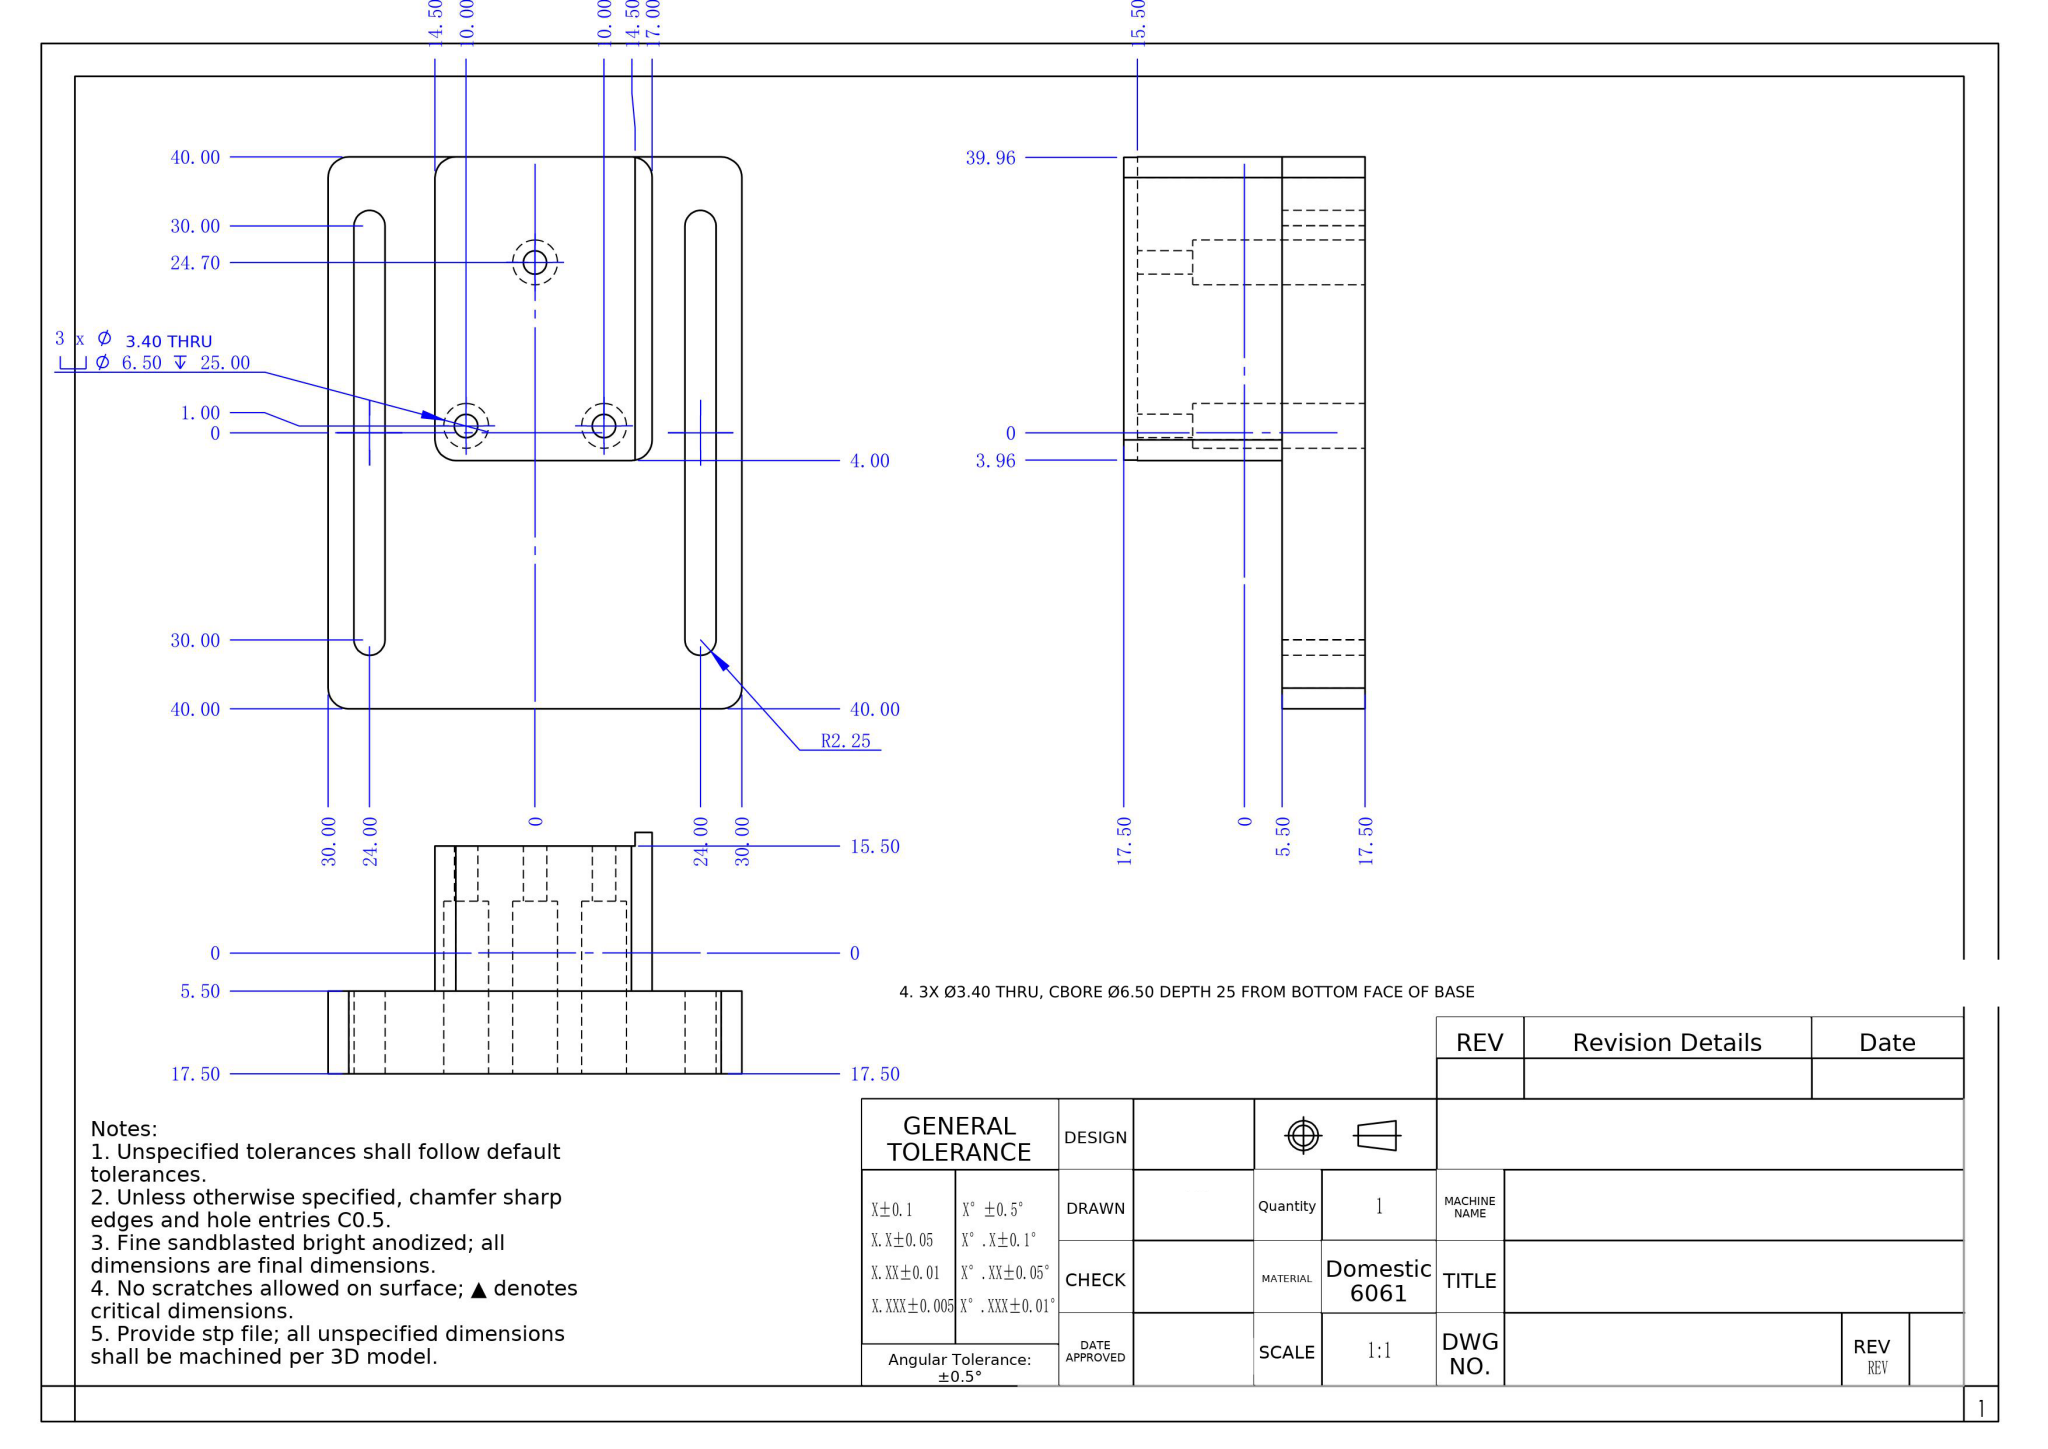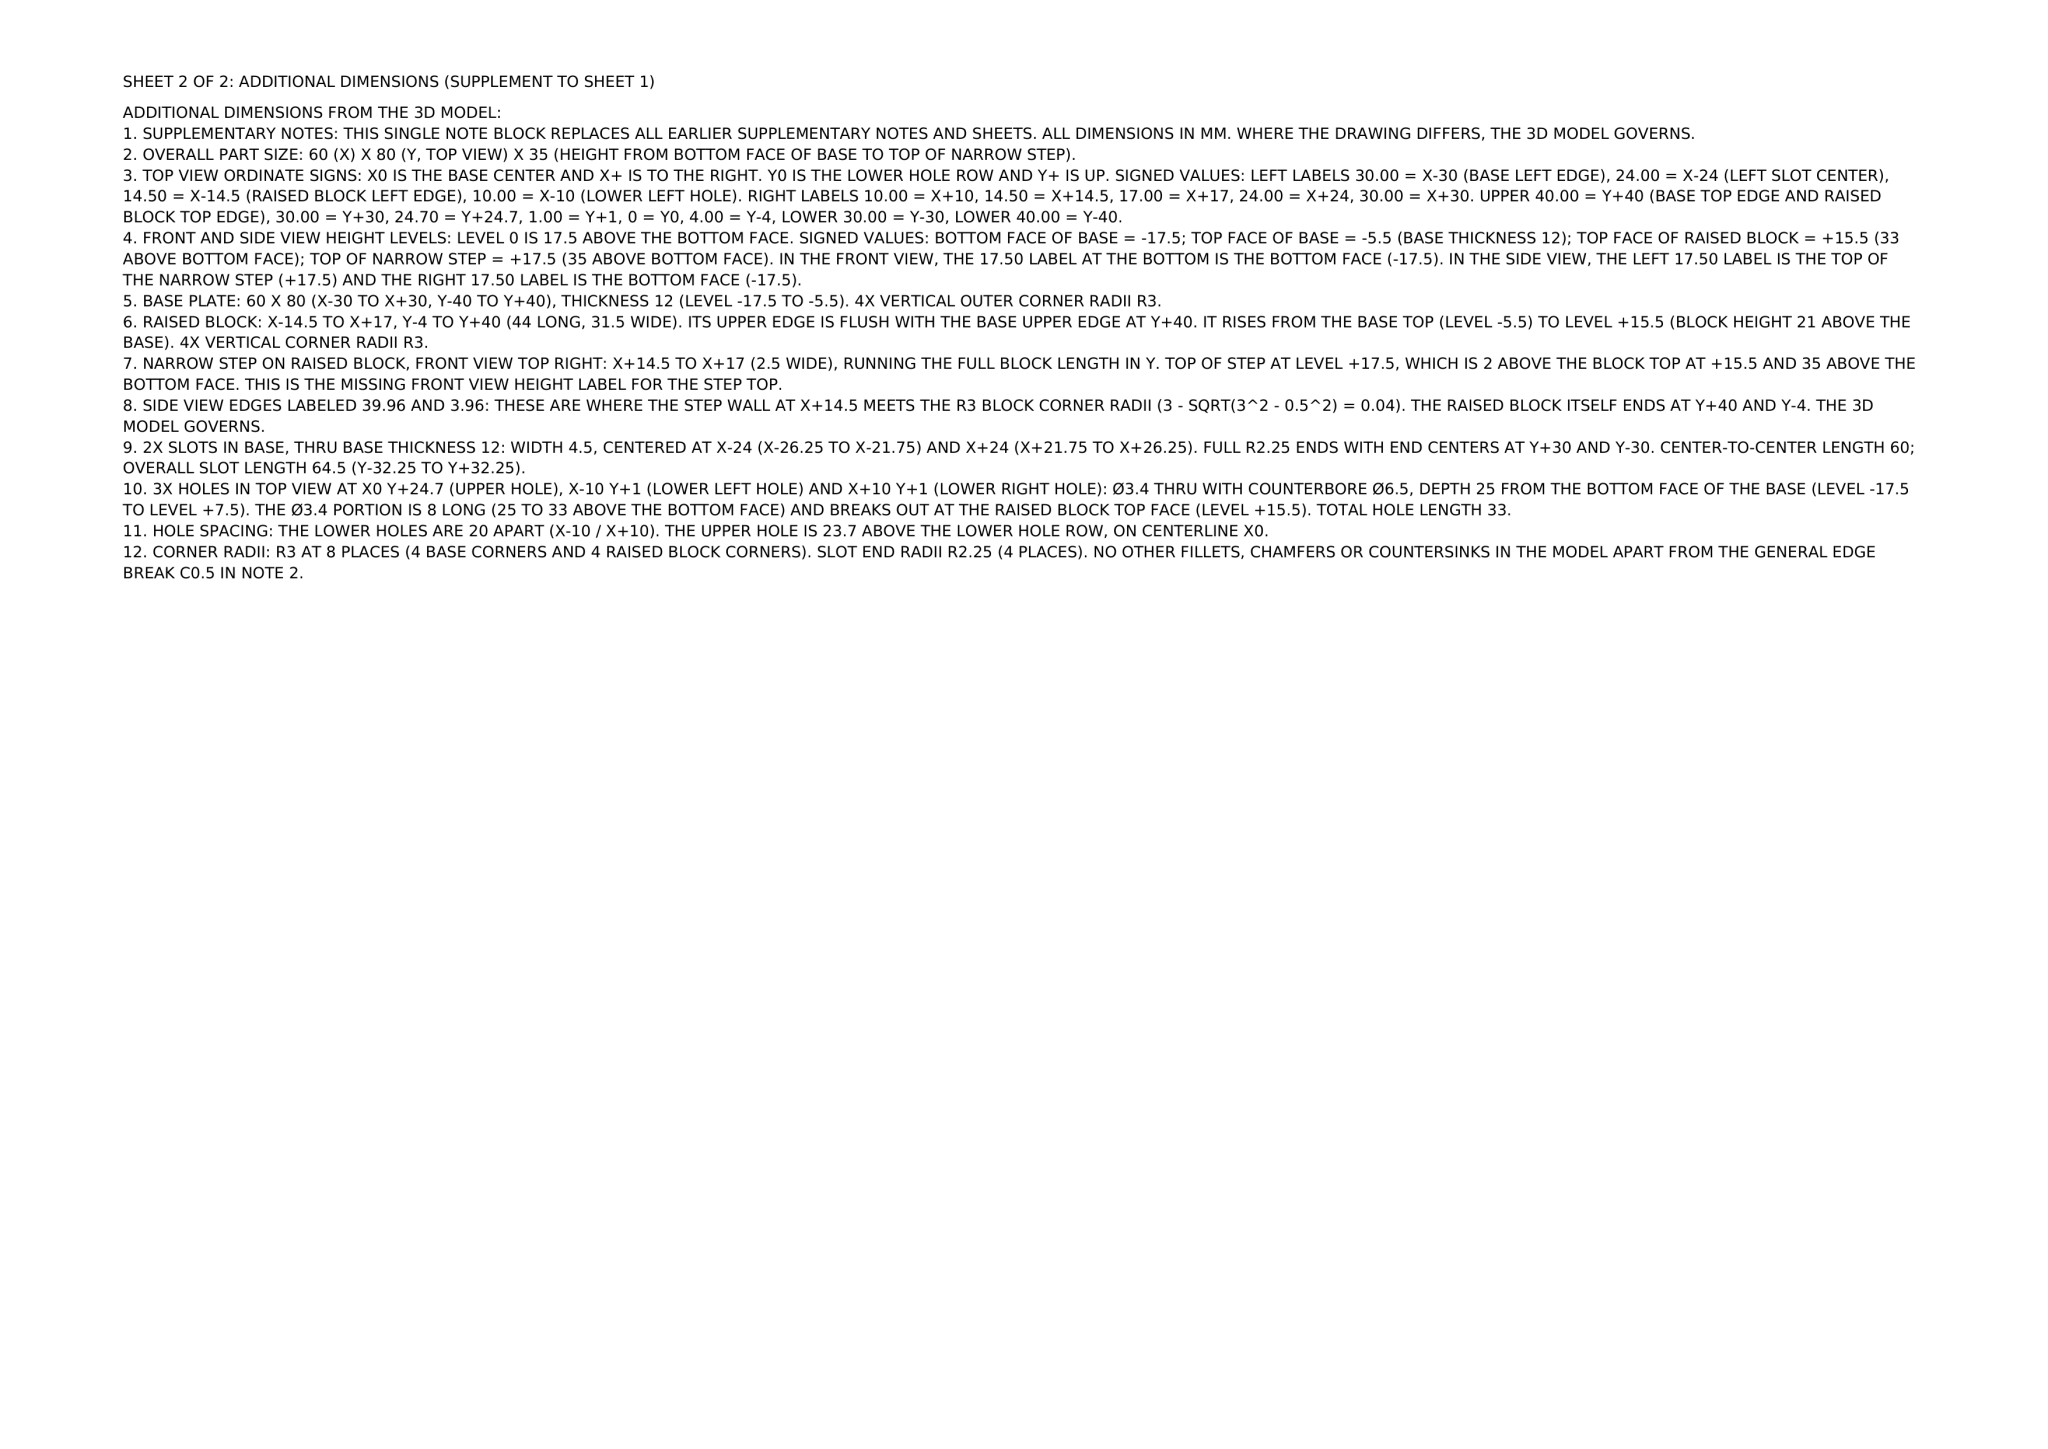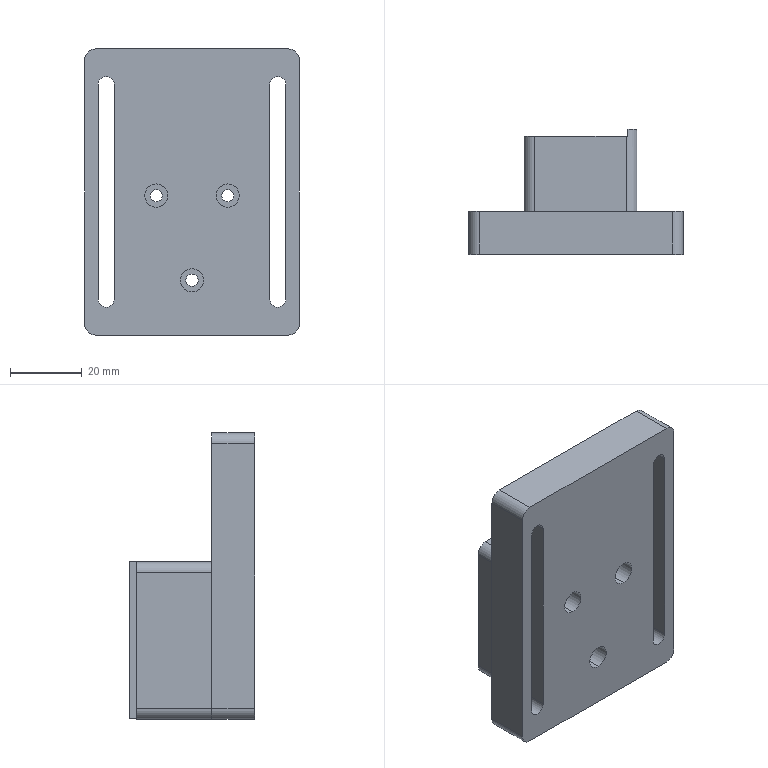Part | NX | mm | 1 solid | 45 faces | box 60 x 35 x 80 mm | volume 77095 mm3 | cylinder 26 | plane 19 | commonest cylinder face diameters 6 x8 4.5 x6 6.5 x6 3.4 x6